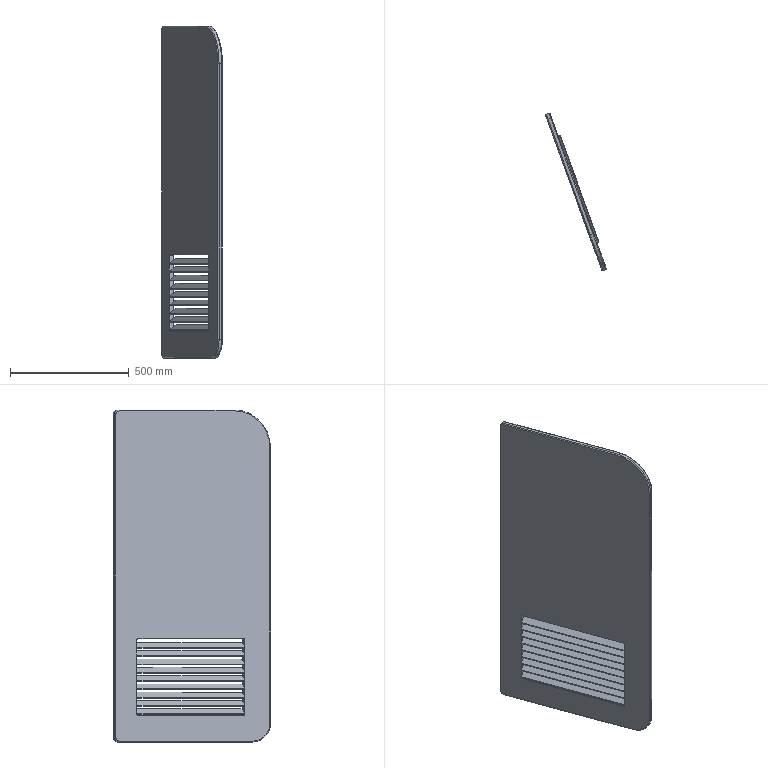Component | NX | DOOR | 10 solids | 106 faces | volume 16742993 mm3 | plane 64 | cylinder 34 | torus 8 | commonest cylinder face diameters 18 x18 8 x8 9 x4 40 x2 160 x1 320 x1